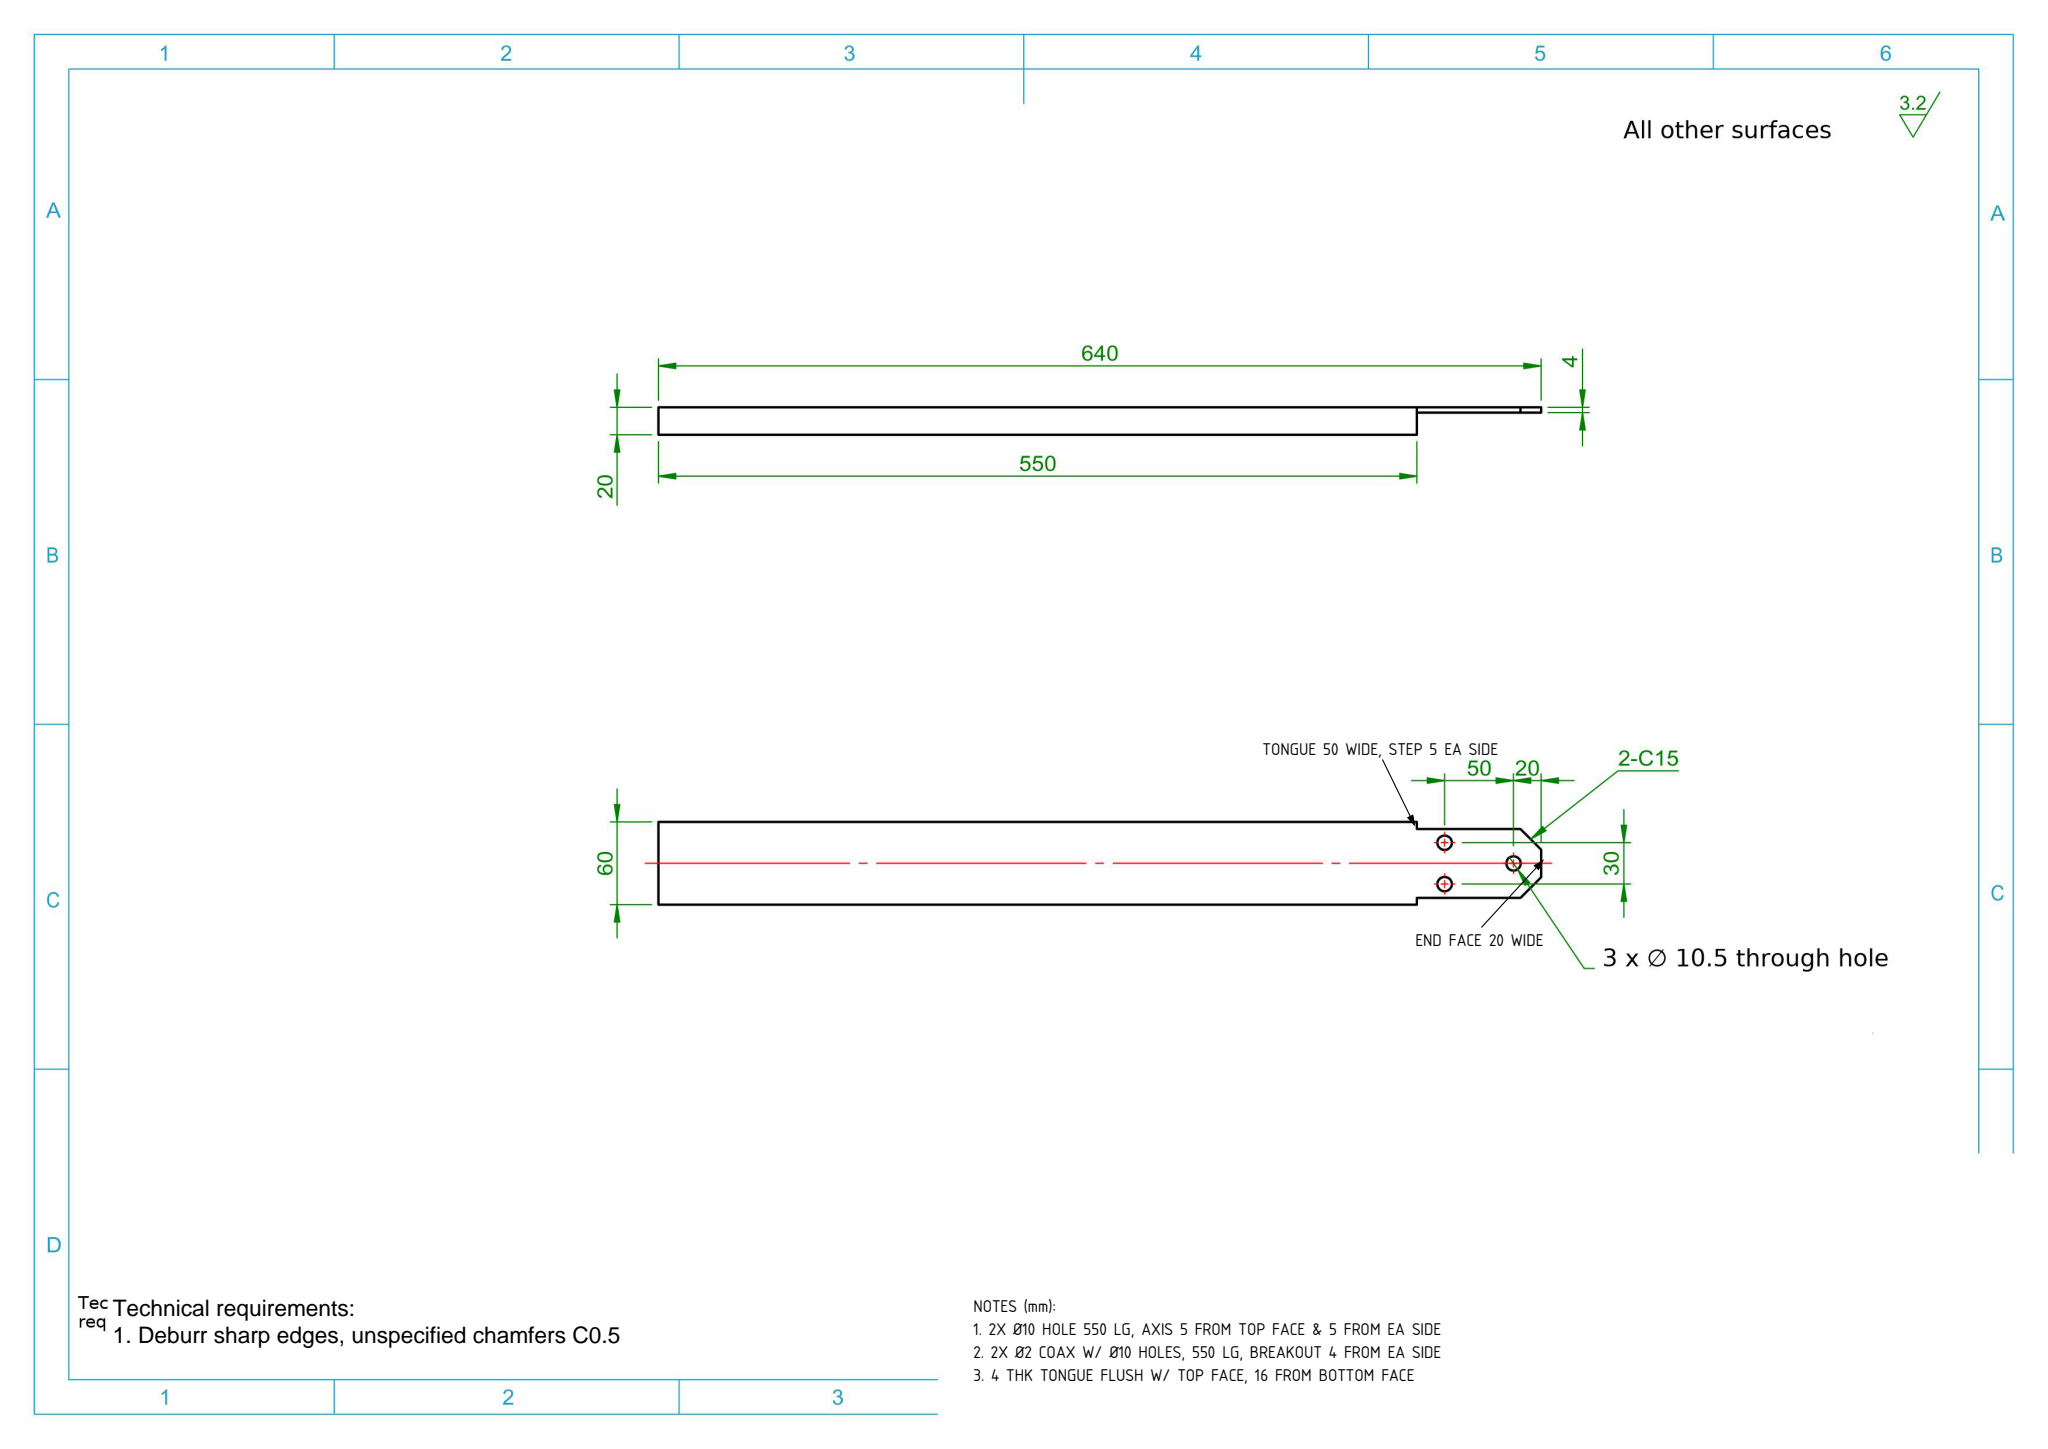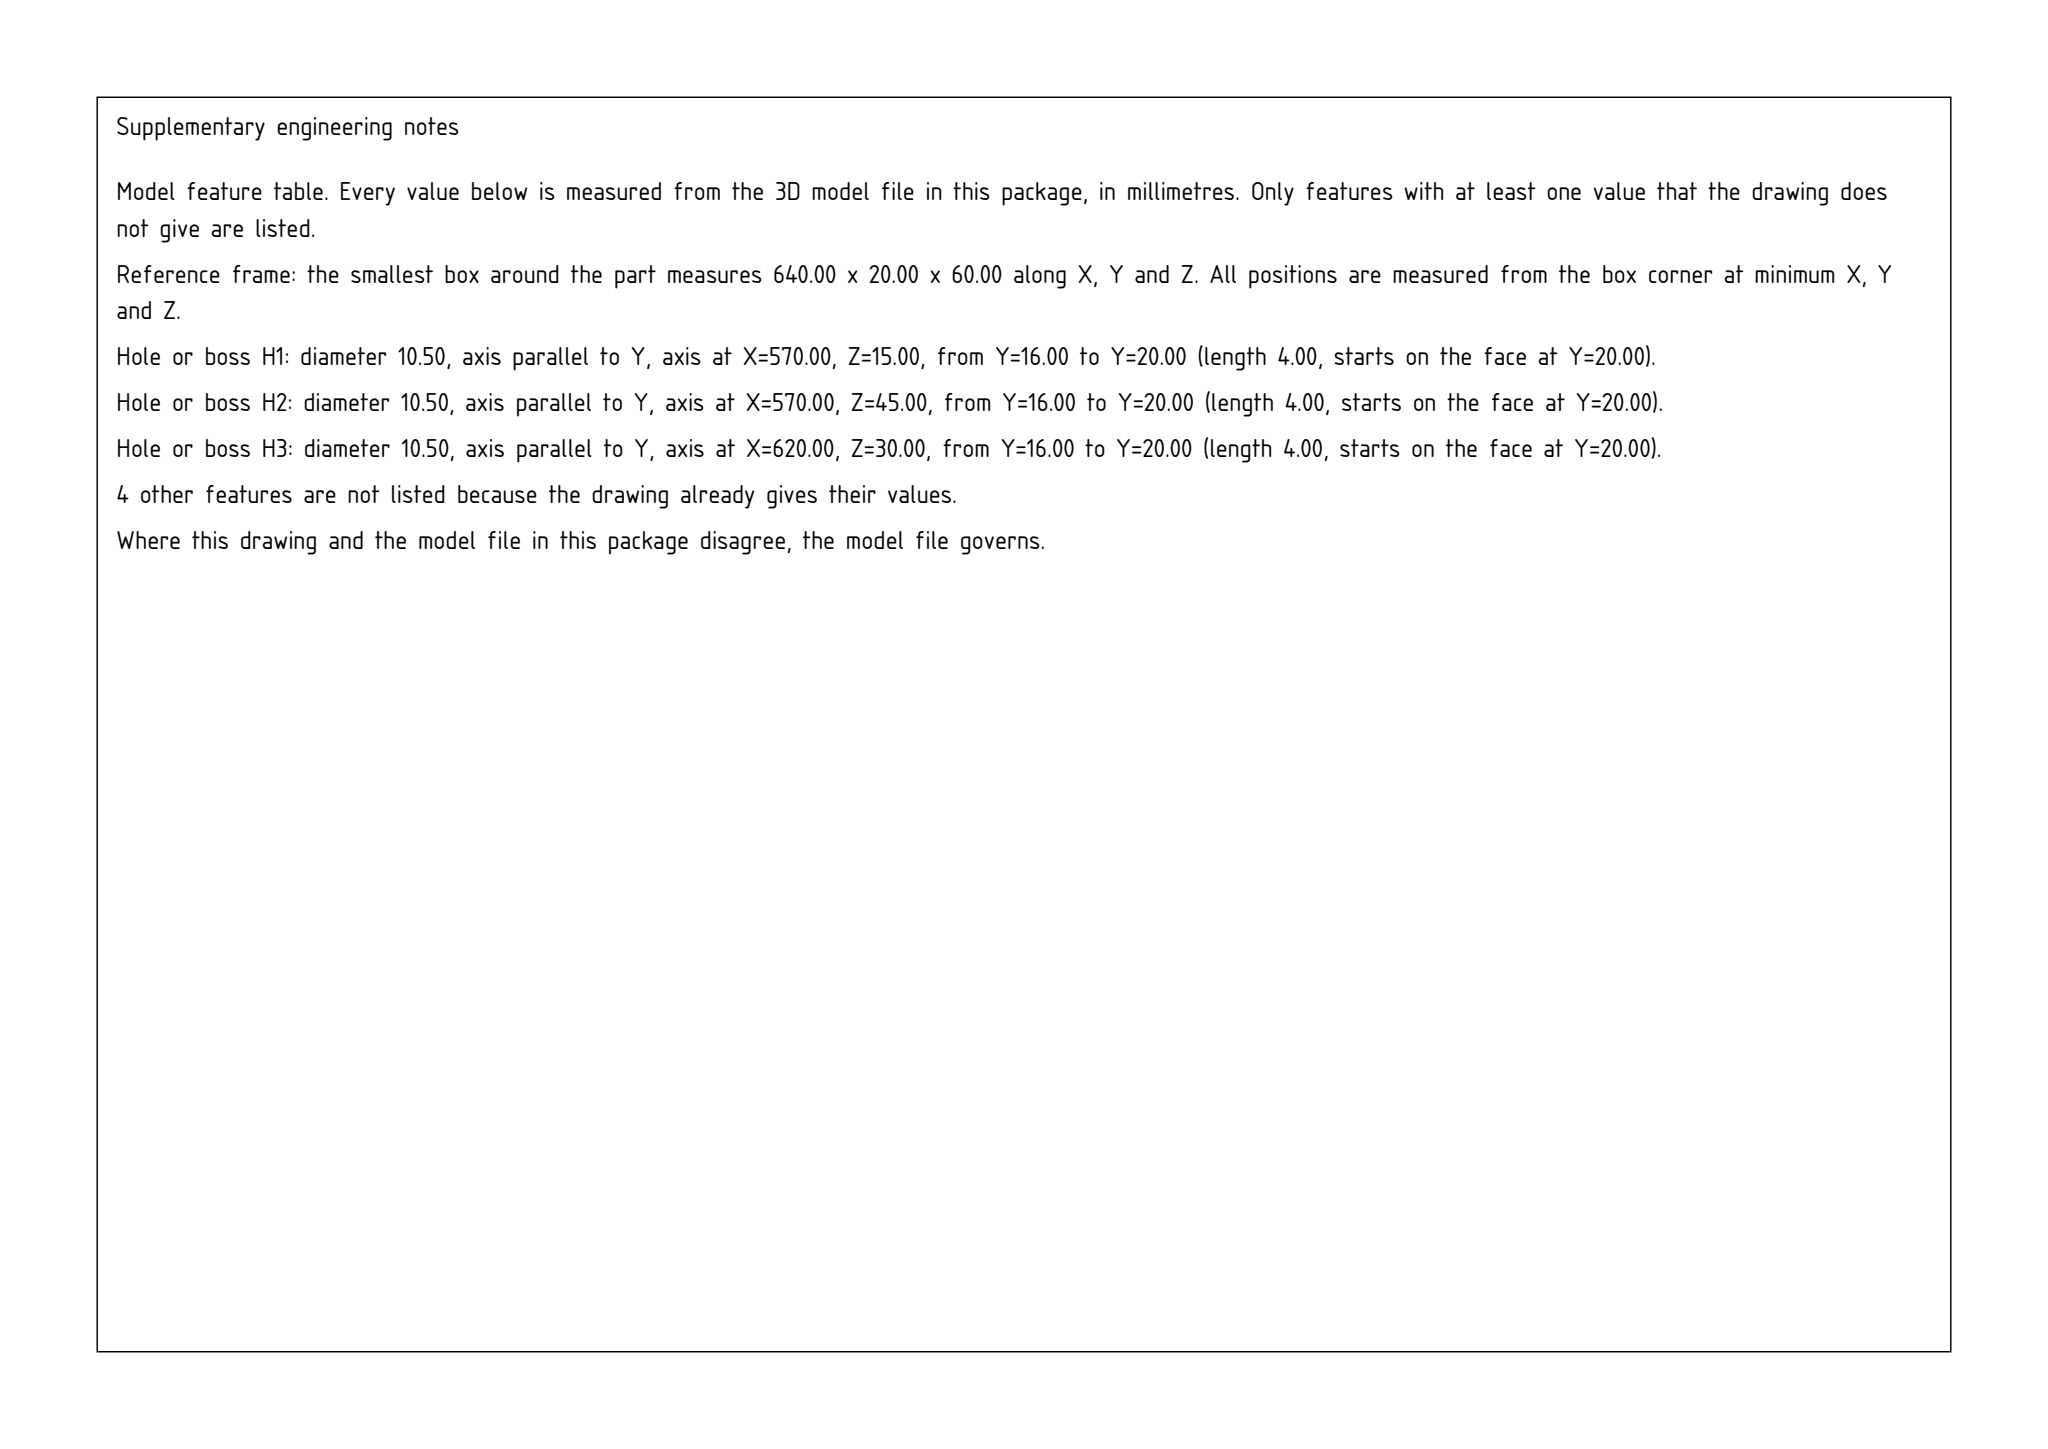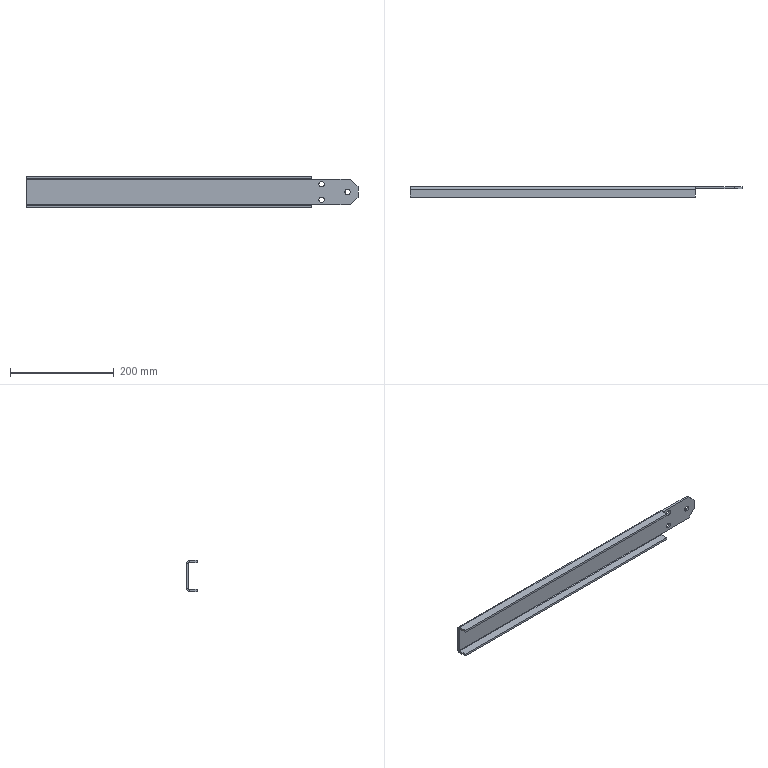Part | SolidWorks | mm | 1 solid | 32 faces | box 640 x 20 x 60 mm | volume 212795 mm3 | plane 22 | cylinder 10 | commonest cylinder face diameters 10.5 x6 10 x2 2 x2
Drawing notes:
TONGUE 50 WIDE (90 LG), STEP 5 DEEP EA SIDE, SYM ABT CL | from the solid: Tongue faces at z=5 and z=55 vs body z=0/60; step at x=550 to x=640
END FACE 20 WIDE AFTER 2-C15, SYM ABT CL | from the solid: 50 wide tongue less 2 x 15 chamfer = 20 at x=640 face
2X Ø10 HOLE 550 LG, AXIS 5 FROM TOP FACE & 5 FROM EA SIDE | from the solid: Ø10 cyl, axis x, y=15 (5 below top y=20), z=5 & z=55, length 550 from x=0
2X Ø2 COAX W/ Ø10 HOLES, 550 LG, BREAKOUT 4 FROM EA SIDE | from the solid: Ø2 cyl, axis x, y=15, z=5 & z=55, L=550; tangent planes z=4 and z=56
4 THK TONGUE FLUSH W/ TOP FACE, 16 FROM BOTTOM FACE | from the solid: y planes at 16 and 20; tongue y=16-20 within 20 thk
STEP:
#1=CARTESIAN_POINT('',(620.,16.,-35.25));
#2=VERTEX_POINT('',#1);
#3=CARTESIAN_POINT('',(620.,16.,-24.75));
#4=VERTEX_POINT('',#3);
#5=CARTESIAN_POINT('',(620.,16.,-30.));
#6=DIRECTION('',(-0.,1.,0.));
#7=DIRECTION('',(0.,0.,1.));
#8=AXIS2_PLACEMENT_3D('',#5,#6,#7);
#9=CIRCLE('',#8,5.25);
#10=EDGE_CURVE('',#2,#4,#9,.T.);
#11=ORIENTED_EDGE('',*,*,#10,.F.);
#12=CARTESIAN_POINT('',(620.,20.,-35.25));
#13=VERTEX_POINT('',#12);
#14=CARTESIAN_POINT('',(620.,20.,-35.25));
#15=DIRECTION('',(-0.,1.,0.));
#16=VECTOR('',#15,1000.);
#17=LINE('',#14,#16);
#18=EDGE_CURVE('',#2,#13,#17,.T.);
#19=ORIENTED_EDGE('',*,*,#18,.T.);
#20=CARTESIAN_POINT('',(620.,20.,-24.75));
#21=VERTEX_POINT('',#20);
#22=CARTESIAN_POINT('',(620.,20.,-30.));
#23=DIRECTION('',(-0.,1.,0.));
#24=DIRECTION('',(0.,0.,1.));
#25=AXIS2_PLACEMENT_3D('',#22,#23,#24);
#26=CIRCLE('',#25,5.25);
#27=EDGE_CURVE('',#13,#21,#26,.T.);
#28=ORIENTED_EDGE('',*,*,#27,.T.);
#29=CARTESIAN_POINT('',(620.,20.,-24.75));
#30=DIRECTION('',(-0.,1.,0.));
#31=VECTOR('',#30,1000.);
#32=LINE('',#29,#31);
#33=EDGE_CURVE('',#4,#21,#32,.T.);
#34=ORIENTED_EDGE('',*,*,#33,.F.);
#35=EDGE_LOOP('',(#11,#19,#28,#34));
#36=FACE_OUTER_BOUND('',#35,.T.);
#37=CARTESIAN_POINT('',(620.,20.,-30.));
#38=DIRECTION('',(-0.,1.,0.));
#39=DIRECTION('',(0.,0.,1.));
#40=AXIS2_PLACEMENT_3D('',#37,#38,#39);
#41=CYLINDRICAL_SURFACE('',#40,5.25);
#42=ADVANCED_FACE('',(#36),#41,.F.);
#43=CARTESIAN_POINT('',(570.,16.,-50.25));
#44=VERTEX_POINT('',#43);
#45=CARTESIAN_POINT('',(570.,16.,-39.75));
#46=VERTEX_POINT('',#45);
#47=CARTESIAN_POINT('',(570.,16.,-45.));
#48=DIRECTION('',(-0.,1.,0.));
#49=DIRECTION('',(0.,0.,1.));
#50=AXIS2_PLACEMENT_3D('',#47,#48,#49);
#51=CIRCLE('',#50,5.25);
#52=EDGE_CURVE('',#44,#46,#51,.T.);
#53=ORIENTED_EDGE('',*,*,#52,.F.);
#54=CARTESIAN_POINT('',(570.,20.,-50.25));
#55=VERTEX_POINT('',#54);
#56=CARTESIAN_POINT('',(570.,20.,-50.25));
#57=DIRECTION('',(-0.,1.,0.));
#58=VECTOR('',#57,1000.);
#59=LINE('',#56,#58);
#60=EDGE_CURVE('',#44,#55,#59,.T.);
#61=ORIENTED_EDGE('',*,*,#60,.T.);
#62=CARTESIAN_POINT('',(570.,20.,-39.75));
#63=VERTEX_POINT('',#62);
#64=CARTESIAN_POINT('',(570.,20.,-45.));
#65=DIRECTION('',(-0.,1.,0.));
#66=DIRECTION('',(0.,0.,1.));
#67=AXIS2_PLACEMENT_3D('',#64,#65,#66);
#68=CIRCLE('',#67,5.25);
#69=EDGE_CURVE('',#55,#63,#68,.T.);
#70=ORIENTED_EDGE('',*,*,#69,.T.);
#71=CARTESIAN_POINT('',(570.,20.,-39.75));
#72=DIRECTION('',(-0.,1.,0.));
#73=VECTOR('',#72,1000.);
#74=LINE('',#71,#73);
#75=EDGE_CURVE('',#46,#63,#74,.T.);
#76=ORIENTED_EDGE('',*,*,#75,.F.);
#77=EDGE_LOOP('',(#53,#61,#70,#76));
#78=FACE_OUTER_BOUND('',#77,.T.);
#79=CARTESIAN_POINT('',(570.,20.,-45.));
#80=DIRECTION('',(-0.,1.,0.));
#81=DIRECTION('',(0.,0.,1.));
#82=AXIS2_PLACEMENT_3D('',#79,#80,#81);
#83=CYLINDRICAL_SURFACE('',#82,5.25);
#84=ADVANCED_FACE('',(#78),#83,.F.);
#85=CARTESIAN_POINT('',(570.,16.,-20.25));
#86=VERTEX_POINT('',#85);
#87=CARTESIAN_POINT('',(570.,16.,-9.75));
#88=VERTEX_POINT('',#87);
#89=CARTESIAN_POINT('',(570.,16.,-15.));
#90=DIRECTION('',(-0.,1.,0.));
#91=DIRECTION('',(0.,0.,1.));
#92=AXIS2_PLACEMENT_3D('',#89,#90,#91);
#93=CIRCLE('',#92,5.25);
#94=EDGE_CURVE('',#86,#88,#93,.T.);
#95=ORIENTED_EDGE('',*,*,#94,.F.);
#96=CARTESIAN_POINT('',(570.,20.,-20.25));
#97=VERTEX_POINT('',#96);
#98=CARTESIAN_POINT('',(570.,20.,-20.25));
#99=DIRECTION('',(-0.,1.,0.));
#100=VECTOR('',#99,1000.);
#101=LINE('',#98,#100);
#102=EDGE_CURVE('',#86,#97,#101,.T.);
#103=ORIENTED_EDGE('',*,*,#102,.T.);
#104=CARTESIAN_POINT('',(570.,20.,-9.75));
#105=VERTEX_POINT('',#104);
#106=CARTESIAN_POINT('',(570.,20.,-15.));
#107=DIRECTION('',(-0.,1.,0.));
#108=DIRECTION('',(0.,0.,1.));
#109=AXIS2_PLACEMENT_3D('',#106,#107,#108);
#110=CIRCLE('',#109,5.25);
#111=EDGE_CURVE('',#97,#105,#110,.T.);
#112=ORIENTED_EDGE('',*,*,#111,.T.);
#113=CARTESIAN_POINT('',(570.,20.,-9.75));
#114=DIRECTION('',(-0.,1.,0.));
#115=VECTOR('',#114,1000.);
#116=LINE('',#113,#115);
#117=EDGE_CURVE('',#88,#105,#116,.T.);
#118=ORIENTED_EDGE('',*,*,#117,.F.);
#119=EDGE_LOOP('',(#95,#103,#112,#118));
#120=FACE_OUTER_BOUND('',#119,.T.);
#121=CARTESIAN_POINT('',(570.,20.,-15.));
#122=DIRECTION('',(-0.,1.,0.));
#123=DIRECTION('',(0.,0.,1.));
#124=AXIS2_PLACEMENT_3D('',#121,#122,#123);
#125=CYLINDRICAL_SURFACE('',#124,5.25);
#126=ADVANCED_FACE('',(#120),#125,.F.);
#127=CARTESIAN_POINT('',(550.,0.,-56.));
#128=VERTEX_POINT('',#127);
#129=CARTESIAN_POINT('',(550.,15.,-56.));
#130=VERTEX_POINT('',#129);
#131=CARTESIAN_POINT('',(550.,0.,-56.));
#132=DIRECTION('',(-0.,1.,0.));
#133=VECTOR('',#132,1000.);
#134=LINE('',#131,#133);
#135=EDGE_CURVE('',#128,#130,#134,.T.);
#136=ORIENTED_EDGE('',*,*,#135,.T.);
#137=CARTESIAN_POINT('',(0.,15.,-56.));
#138=VERTEX_POINT('',#137);
#139=CARTESIAN_POINT('',(640.,15.,-56.));
#140=DIRECTION('',(-1.,0.,0.));
#141=VECTOR('',#140,1000.);
#142=LINE('',#139,#141);
#143=EDGE_CURVE('',#130,#138,#142,.T.);
#144=ORIENTED_EDGE('',*,*,#143,.T.);
#145=CARTESIAN_POINT('',(0.,0.,-56.));
#146=VERTEX_POINT('',#145);
#147=CARTESIAN_POINT('',(0.,20.,-56.));
#148=DIRECTION('',(0.,-1.,-0.));
#149=VECTOR('',#148,1000.);
#150=LINE('',#147,#149);
#151=EDGE_CURVE('',#138,#146,#150,.T.);
#152=ORIENTED_EDGE('',*,*,#151,.T.);
#153=CARTESIAN_POINT('',(640.,0.,-56.));
#154=DIRECTION('',(-1.,0.,0.));
#155=VECTOR('',#154,1000.);
#156=LINE('',#153,#155);
#157=EDGE_CURVE('',#128,#146,#156,.T.);
#158=ORIENTED_EDGE('',*,*,#157,.F.);
#159=EDGE_LOOP('',(#136,#144,#152,#158));
#160=FACE_OUTER_BOUND('',#159,.T.);
#161=CARTESIAN_POINT('',(640.,20.,-56.));
#162=DIRECTION('',(-0.,-0.,-1.));
#163=DIRECTION('',(-1.,0.,0.));
#164=AXIS2_PLACEMENT_3D('',#161,#162,#163);
#165=PLANE('',#164);
#166=ADVANCED_FACE('',(#160),#165,.F.);
#167=CARTESIAN_POINT('',(550.,0.,-60.));
#168=VERTEX_POINT('',#167);
#169=CARTESIAN_POINT('',(0.,0.,-60.));
#170=VERTEX_POINT('',#169);
#171=CARTESIAN_POINT('',(640.,0.,-60.));
#172=DIRECTION('',(-1.,0.,0.));
#173=VECTOR('',#172,1000.);
#174=LINE('',#171,#173);
#175=EDGE_CURVE('',#168,#170,#174,.T.);
#176=ORIENTED_EDGE('',*,*,#175,.F.);
#177=CARTESIAN_POINT('',(550.,0.,-56.));
#178=DIRECTION('',(-0.,0.,1.));
#179=VECTOR('',#178,1000.);
#180=LINE('',#177,#179);
#181=EDGE_CURVE('',#168,#128,#180,.T.);
#182=ORIENTED_EDGE('',*,*,#181,.T.);
#183=ORIENTED_EDGE('',*,*,#157,.T.);
#184=CARTESIAN_POINT('',(0.,0.,-60.));
#185=DIRECTION('',(-0.,0.,1.));
#186=VECTOR('',#185,1000.);
#187=LINE('',#184,#186);
#188=EDGE_CURVE('',#170,#146,#187,.T.);
#189=ORIENTED_EDGE('',*,*,#188,.F.);
#190=EDGE_LOOP('',(#176,#182,#183,#189));
#191=FACE_OUTER_BOUND('',#190,.T.);
#192=CARTESIAN_POINT('',(640.,0.,-60.));
#193=DIRECTION('',(0.,-1.,0.));
#194=DIRECTION('',(0.,-0.,-1.));
#195=AXIS2_PLACEMENT_3D('',#192,#193,#194);
#196=PLANE('',#195);
#197=ADVANCED_FACE('',(#191),#196,.T.);
#198=CARTESIAN_POINT('',(550.,15.,-60.));
#199=VERTEX_POINT('',#198);
#200=CARTESIAN_POINT('',(0.,15.,-60.));
#201=VERTEX_POINT('',#200);
#202=CARTESIAN_POINT('',(640.,15.,-60.));
#203=DIRECTION('',(-1.,0.,0.));
#204=VECTOR('',#203,1000.);
#205=LINE('',#202,#204);
#206=EDGE_CURVE('',#199,#201,#205,.T.);
#207=ORIENTED_EDGE('',*,*,#206,.F.);
#208=CARTESIAN_POINT('',(550.,7.5,-60.));
#209=DIRECTION('',(-0.,1.,0.));
#210=VECTOR('',#209,1000.);
#211=LINE('',#208,#210);
#212=EDGE_CURVE('',#168,#199,#211,.T.);
#213=ORIENTED_EDGE('',*,*,#212,.F.);
#214=ORIENTED_EDGE('',*,*,#175,.T.);
#215=CARTESIAN_POINT('',(0.,20.,-60.));
#216=DIRECTION('',(0.,-1.,-0.));
#217=VECTOR('',#216,1000.);
#218=LINE('',#215,#217);
#219=EDGE_CURVE('',#201,#170,#218,.T.);
#220=ORIENTED_EDGE('',*,*,#219,.F.);
#221=EDGE_LOOP('',(#207,#213,#214,#220));
#222=FACE_OUTER_BOUND('',#221,.T.);
#223=CARTESIAN_POINT('',(640.,20.,-60.));
#224=DIRECTION('',(-0.,-0.,-1.));
#225=DIRECTION('',(-1.,0.,0.));
#226=AXIS2_PLACEMENT_3D('',#223,#224,#225);
#227=PLANE('',#226);
#228=ADVANCED_FACE('',(#222),#227,.T.);
#229=CARTESIAN_POINT('',(550.,20.,-55.));
#230=VERTEX_POINT('',#229);
#231=CARTESIAN_POINT('',(0.,20.,-55.));
#232=VERTEX_POINT('',#231);
#233=CARTESIAN_POINT('',(640.,20.,-55.));
#234=DIRECTION('',(-1.,0.,0.));
#235=VECTOR('',#234,1000.);
#236=LINE('',#233,#235);
#237=EDGE_CURVE('',#230,#232,#236,.T.);
#238=ORIENTED_EDGE('',*,*,#237,.F.);
#239=CARTESIAN_POINT('',(550.,15.,-55.));
#240=DIRECTION('',(-1.,0.,0.));
#241=DIRECTION('',(0.,0.,1.));
#242=AXIS2_PLACEMENT_3D('',#239,#240,#241);
#243=CIRCLE('',#242,5.);
#244=EDGE_CURVE('',#230,#199,#243,.T.);
#245=ORIENTED_EDGE('',*,*,#244,.T.);
#246=ORIENTED_EDGE('',*,*,#206,.T.);
#247=CARTESIAN_POINT('',(0.,15.,-55.));
#248=DIRECTION('',(-1.,0.,0.));
#249=DIRECTION('',(0.,0.,-1.));
#250=AXIS2_PLACEMENT_3D('',#247,#248,#249);
#251=CIRCLE('',#250,5.);
#252=EDGE_CURVE('',#232,#201,#251,.T.);
#253=ORIENTED_EDGE('',*,*,#252,.F.);
#254=EDGE_LOOP('',(#238,#245,#246,#253));
#255=FACE_OUTER_BOUND('',#254,.T.);
#256=CARTESIAN_POINT('',(640.,15.,-55.));
#257=DIRECTION('',(-1.,0.,0.));
#258=DIRECTION('',(0.,0.,1.));
#259=AXIS2_PLACEMENT_3D('',#256,#257,#258);
#260=CYLINDRICAL_SURFACE('',#259,5.);
#261=ADVANCED_FACE('',(#255),#260,.T.);
#262=CARTESIAN_POINT('',(550.,15.,-0.));
#263=VERTEX_POINT('',#262);
#264=CARTESIAN_POINT('',(0.,15.,0.));
#265=VERTEX_POINT('',#264);
#266=CARTESIAN_POINT('',(640.,15.,-0.));
#267=DIRECTION('',(-1.,0.,0.));
#268=VECTOR('',#267,1000.);
#269=LINE('',#266,#268);
#270=EDGE_CURVE('',#263,#265,#269,.T.);
#271=ORIENTED_EDGE('',*,*,#270,.F.);
#272=CARTESIAN_POINT('',(550.,20.,-5.));
#273=VERTEX_POINT('',#272);
#274=CARTESIAN_POINT('',(550.,15.,-5.));
#275=DIRECTION('',(-1.,0.,0.));
#276=DIRECTION('',(0.,0.,1.));
#277=AXIS2_PLACEMENT_3D('',#274,#275,#276);
#278=CIRCLE('',#277,5.);
#279=EDGE_CURVE('',#263,#273,#278,.T.);
#280=ORIENTED_EDGE('',*,*,#279,.T.);
#281=CARTESIAN_POINT('',(0.,20.,-5.));
#282=VERTEX_POINT('',#281);
#283=CARTESIAN_POINT('',(640.,20.,-5.));
#284=DIRECTION('',(-1.,0.,0.));
#285=VECTOR('',#284,1000.);
#286=LINE('',#283,#285);
#287=EDGE_CURVE('',#273,#282,#286,.T.);
#288=ORIENTED_EDGE('',*,*,#287,.T.);
#289=CARTESIAN_POINT('',(0.,15.,-5.));
#290=DIRECTION('',(-1.,0.,0.));
#291=DIRECTION('',(0.,0.,-1.));
#292=AXIS2_PLACEMENT_3D('',#289,#290,#291);
#293=CIRCLE('',#292,5.);
#294=EDGE_CURVE('',#265,#282,#293,.T.);
#295=ORIENTED_EDGE('',*,*,#294,.F.);
#296=EDGE_LOOP('',(#271,#280,#288,#295));
#297=FACE_OUTER_BOUND('',#296,.T.);
#298=CARTESIAN_POINT('',(640.,15.,-5.));
#299=DIRECTION('',(-1.,0.,0.));
#300=DIRECTION('',(0.,0.,1.));
#301=AXIS2_PLACEMENT_3D('',#298,#299,#300);
#302=CYLINDRICAL_SURFACE('',#301,5.);
#303=ADVANCED_FACE('',(#297),#302,.T.);
#304=CARTESIAN_POINT('',(550.,-0.,-0.));
#305=VERTEX_POINT('',#304);
#306=CARTESIAN_POINT('',(0.,0.,0.));
#307=VERTEX_POINT('',#306);
#308=CARTESIAN_POINT('',(640.,0.,-0.));
#309=DIRECTION('',(-1.,0.,0.));
#310=VECTOR('',#309,1000.);
#311=LINE('',#308,#310);
#312=EDGE_CURVE('',#305,#307,#311,.T.);
#313=ORIENTED_EDGE('',*,*,#312,.F.);
#314=CARTESIAN_POINT('',(550.,-0.,-0.));
#315=DIRECTION('',(-0.,1.,0.));
#316=VECTOR('',#315,1000.);
#317=LINE('',#314,#316);
#318=EDGE_CURVE('',#305,#263,#317,.T.);
#319=ORIENTED_EDGE('',*,*,#318,.T.);
#320=ORIENTED_EDGE('',*,*,#270,.T.);
#321=CARTESIAN_POINT('',(0.,0.,0.));
#322=DIRECTION('',(-0.,1.,0.));
#323=VECTOR('',#322,1000.);
#324=LINE('',#321,#323);
#325=EDGE_CURVE('',#307,#265,#324,.T.);
#326=ORIENTED_EDGE('',*,*,#325,.F.);
#327=EDGE_LOOP('',(#313,#319,#320,#326));
#328=FACE_OUTER_BOUND('',#327,.T.);
#329=CARTESIAN_POINT('',(640.,0.,-0.));
#330=DIRECTION('',(0.,0.,1.));
#331=DIRECTION('',(1.,-0.,-0.));
#332=AXIS2_PLACEMENT_3D('',#329,#330,#331);
#333=PLANE('',#332);
#334=ADVANCED_FACE('',(#328),#333,.T.);
#335=CARTESIAN_POINT('',(550.,0.,-4.));
#336=VERTEX_POINT('',#335);
#337=CARTESIAN_POINT('',(0.,0.,-4.));
#338=VERTEX_POINT('',#337);
#339=CARTESIAN_POINT('',(640.,0.,-4.));
#340=DIRECTION('',(-1.,0.,0.));
#341=VECTOR('',#340,1000.);
#342=LINE('',#339,#341);
#343=EDGE_CURVE('',#336,#338,#342,.T.);
#344=ORIENTED_EDGE('',*,*,#343,.F.);
#345=CARTESIAN_POINT('',(550.,-0.,-0.));
#346=DIRECTION('',(-0.,0.,1.));
#347=VECTOR('',#346,1000.);
#348=LINE('',#345,#347);
#349=EDGE_CURVE('',#336,#305,#348,.T.);
#350=ORIENTED_EDGE('',*,*,#349,.T.);
#351=ORIENTED_EDGE('',*,*,#312,.T.);
#352=CARTESIAN_POINT('',(0.,0.,-4.));
#353=DIRECTION('',(-0.,0.,1.));
#354=VECTOR('',#353,1000.);
#355=LINE('',#352,#354);
#356=EDGE_CURVE('',#338,#307,#355,.T.);
#357=ORIENTED_EDGE('',*,*,#356,.F.);
#358=EDGE_LOOP('',(#344,#350,#351,#357));
#359=FACE_OUTER_BOUND('',#358,.T.);
#360=CARTESIAN_POINT('',(640.,0.,-4.));
#361=DIRECTION('',(0.,-1.,0.));
#362=DIRECTION('',(0.,-0.,-1.));
#363=AXIS2_PLACEMENT_3D('',#360,#361,#362);
#364=PLANE('',#363);
#365=ADVANCED_FACE('',(#359),#364,.T.);
#366=CARTESIAN_POINT('',(550.,15.,-4.));
#367=VERTEX_POINT('',#366);
#368=CARTESIAN_POINT('',(550.,7.5,-4.));
#369=DIRECTION('',(-0.,1.,0.));
#370=VECTOR('',#369,1000.);
#371=LINE('',#368,#370);
#372=EDGE_CURVE('',#336,#367,#371,.T.);
#373=ORIENTED_EDGE('',*,*,#372,.F.);
#374=ORIENTED_EDGE('',*,*,#343,.T.);
#375=CARTESIAN_POINT('',(0.,15.,-4.));
#376=VERTEX_POINT('',#375);
#377=CARTESIAN_POINT('',(0.,0.,-4.));
#378=DIRECTION('',(-0.,1.,0.));
#379=VECTOR('',#378,1000.);
#380=LINE('',#377,#379);
#381=EDGE_CURVE('',#338,#376,#380,.T.);
#382=ORIENTED_EDGE('',*,*,#381,.T.);
#383=CARTESIAN_POINT('',(640.,15.,-4.));
#384=DIRECTION('',(-1.,0.,0.));
#385=VECTOR('',#384,1000.);
#386=LINE('',#383,#385);
#387=EDGE_CURVE('',#367,#376,#386,.T.);
#388=ORIENTED_EDGE('',*,*,#387,.F.);
#389=EDGE_LOOP('',(#373,#374,#382,#388));
#390=FACE_OUTER_BOUND('',#389,.T.);
#391=CARTESIAN_POINT('',(640.,0.,-4.));
#392=DIRECTION('',(0.,0.,1.));
#393=DIRECTION('',(1.,-0.,-0.));
#394=AXIS2_PLACEMENT_3D('',#391,#392,#393);
#395=PLANE('',#394);
#396=ADVANCED_FACE('',(#390),#395,.F.);
#397=CARTESIAN_POINT('',(550.,16.,-5.));
#398=VERTEX_POINT('',#397);
#399=CARTESIAN_POINT('',(550.,15.,-5.));
#400=DIRECTION('',(-1.,0.,0.));
#401=DIRECTION('',(0.,0.,-1.));
#402=AXIS2_PLACEMENT_3D('',#399,#400,#401);
#403=CIRCLE('',#402,1.);
#404=EDGE_CURVE('',#367,#398,#403,.T.);
#405=ORIENTED_EDGE('',*,*,#404,.F.);
#406=ORIENTED_EDGE('',*,*,#387,.T.);
#407=CARTESIAN_POINT('',(0.,16.,-5.));
#408=VERTEX_POINT('',#407);
#409=CARTESIAN_POINT('',(0.,15.,-5.));
#410=DIRECTION('',(-1.,0.,0.));
#411=DIRECTION('',(0.,0.,-1.));
#412=AXIS2_PLACEMENT_3D('',#409,#410,#411);
#413=CIRCLE('',#412,1.);
#414=EDGE_CURVE('',#376,#408,#413,.T.);
#415=ORIENTED_EDGE('',*,*,#414,.T.);
#416=CARTESIAN_POINT('',(640.,16.,-5.));
#417=DIRECTION('',(-1.,0.,0.));
#418=VECTOR('',#417,1000.);
#419=LINE('',#416,#418);
#420=EDGE_CURVE('',#398,#408,#419,.T.);
#421=ORIENTED_EDGE('',*,*,#420,.F.);
#422=EDGE_LOOP('',(#405,#406,#415,#421));
#423=FACE_OUTER_BOUND('',#422,.T.);
#424=CARTESIAN_POINT('',(640.,15.,-5.));
#425=DIRECTION('',(-1.,0.,0.));
#426=DIRECTION('',(0.,0.,1.));
#427=AXIS2_PLACEMENT_3D('',#424,#425,#426);
#428=CYLINDRICAL_SURFACE('',#427,1.);
#429=ADVANCED_FACE('',(#423),#428,.F.);
#430=CARTESIAN_POINT('',(550.,16.,-55.));
#431=VERTEX_POINT('',#430);
#432=CARTESIAN_POINT('',(550.,15.,-55.));
#433=DIRECTION('',(-1.,0.,0.));
#434=DIRECTION('',(0.,0.,1.));
#435=AXIS2_PLACEMENT_3D('',#432,#433,#434);
#436=CIRCLE('',#435,1.);
#437=EDGE_CURVE('',#431,#130,#436,.T.);
#438=ORIENTED_EDGE('',*,*,#437,.F.);
#439=CARTESIAN_POINT('',(0.,16.,-55.));
#440=VERTEX_POINT('',#439);
#441=CARTESIAN_POINT('',(640.,16.,-55.));
#442=DIRECTION('',(-1.,0.,0.));
#443=VECTOR('',#442,1000.);
#444=LINE('',#441,#443);
#445=EDGE_CURVE('',#431,#440,#444,.T.);
#446=ORIENTED_EDGE('',*,*,#445,.T.);
#447=CARTESIAN_POINT('',(0.,15.,-55.));
#448=DIRECTION('',(-1.,0.,0.));
#449=DIRECTION('',(0.,0.,-1.));
#450=AXIS2_PLACEMENT_3D('',#447,#448,#449);
#451=CIRCLE('',#450,1.);
#452=EDGE_CURVE('',#440,#138,#451,.T.);
#453=ORIENTED_EDGE('',*,*,#452,.T.);
#454=ORIENTED_EDGE('',*,*,#143,.F.);
#455=EDGE_LOOP('',(#438,#446,#453,#454));
#456=FACE_OUTER_BOUND('',#455,.T.);
#457=CARTESIAN_POINT('',(640.,15.,-55.));
#458=DIRECTION('',(-1.,0.,0.));
#459=DIRECTION('',(0.,0.,1.));
#460=AXIS2_PLACEMENT_3D('',#457,#458,#459);
#461=CYLINDRICAL_SURFACE('',#460,1.);
#462=ADVANCED_FACE('',(#456),#461,.F.);
#463=CARTESIAN_POINT('',(640.,20.,-20.));
#464=VERTEX_POINT('',#463);
#465=CARTESIAN_POINT('',(640.,20.,-40.));
#466=VERTEX_POINT('',#465);
#467=CARTESIAN_POINT('',(640.,20.,-0.));
#468=DIRECTION('',(0.,-0.,-1.));
#469=VECTOR('',#468,1000.);
#470=LINE('',#467,#469);
#471=EDGE_CURVE('',#464,#466,#470,.T.);
#472=ORIENTED_EDGE('',*,*,#471,.F.);
#473=CARTESIAN_POINT('',(640.,16.,-20.));
#474=VERTEX_POINT('',#473);
#475=CARTESIAN_POINT('',(640.,15.,-20.));
#476=DIRECTION('',(0.,-1.,-0.));
#477=VECTOR('',#476,1000.);
#478=LINE('',#475,#477);
#479=EDGE_CURVE('',#464,#474,#478,.T.);
#480=ORIENTED_EDGE('',*,*,#479,.T.);
#481=CARTESIAN_POINT('',(640.,16.,-40.));
#482=VERTEX_POINT('',#481);
#483=CARTESIAN_POINT('',(640.,16.,-0.));
#484=DIRECTION('',(0.,-0.,-1.));
#485=VECTOR('',#484,1000.);
#486=LINE('',#483,#485);
#487=EDGE_CURVE('',#474,#482,#486,.T.);
#488=ORIENTED_EDGE('',*,*,#487,.T.);
#489=CARTESIAN_POINT('',(640.,15.,-40.));
#490=DIRECTION('',(-0.,1.,0.));
#491=VECTOR('',#490,1000.);
#492=LINE('',#489,#491);
#493=EDGE_CURVE('',#482,#466,#492,.T.);
#494=ORIENTED_EDGE('',*,*,#493,.T.);
#495=EDGE_LOOP('',(#472,#480,#488,#494));
#496=FACE_OUTER_BOUND('',#495,.T.);
#497=CARTESIAN_POINT('',(640.,15.,-4.));
#498=DIRECTION('',(1.,-0.,0.));
#499=DIRECTION('',(0.,-0.,-1.));
#500=AXIS2_PLACEMENT_3D('',#497,#498,#499);
#501=PLANE('',#500);
#502=ADVANCED_FACE('',(#496),#501,.T.);
#503=CARTESIAN_POINT('',(0.,15.,0.));
#504=DIRECTION('',(0.,-0.,-1.));
#505=VECTOR('',#504,1000.);
#506=LINE('',#503,#505);
#507=EDGE_CURVE('',#265,#376,#506,.T.);
#508=ORIENTED_EDGE('',*,*,#507,.F.);
#509=ORIENTED_EDGE('',*,*,#294,.T.);
#510=CARTESIAN_POINT('',(0.,16.,-5.));
#511=DIRECTION('',(-0.,1.,0.));
#512=VECTOR('',#511,1000.);
#513=LINE('',#510,#512);
#514=EDGE_CURVE('',#408,#282,#513,.T.);
#515=ORIENTED_EDGE('',*,*,#514,.F.);
#516=ORIENTED_EDGE('',*,*,#414,.F.);
#517=EDGE_LOOP('',(#508,#509,#515,#516));
#518=FACE_OUTER_BOUND('',#517,.T.);
#519=CARTESIAN_POINT('',(0.,15.,0.));
#520=DIRECTION('',(-1.,0.,-0.));
#521=DIRECTION('',(-0.,0.,1.));
#522=AXIS2_PLACEMENT_3D('',#519,#520,#521);
#523=PLANE('',#522);
#524=ADVANCED_FACE('',(#518),#523,.T.);
#525=ORIENTED_EDGE('',*,*,#325,.T.);
#526=ORIENTED_EDGE('',*,*,#507,.T.);
#527=ORIENTED_EDGE('',*,*,#381,.F.);
#528=ORIENTED_EDGE('',*,*,#356,.T.);
#529=EDGE_LOOP('',(#525,#526,#527,#528));
#530=FACE_OUTER_BOUND('',#529,.T.);
#531=CARTESIAN_POINT('',(0.,16.,-5.));
#532=DIRECTION('',(-1.,0.,-0.));
#533=DIRECTION('',(-0.,0.,1.));
#534=AXIS2_PLACEMENT_3D('',#531,#532,#533);
#535=PLANE('',#534);
#536=ADVANCED_FACE('',(#530),#535,.T.);
#537=CARTESIAN_POINT('',(0.,20.,-55.));
#538=DIRECTION('',(0.,-1.,-0.));
#539=VECTOR('',#538,1000.);
#540=LINE('',#537,#539);
#541=EDGE_CURVE('',#232,#440,#540,.T.);
#542=ORIENTED_EDGE('',*,*,#541,.F.);
#543=ORIENTED_EDGE('',*,*,#252,.T.);
#544=CARTESIAN_POINT('',(0.,15.,-56.));
#545=DIRECTION('',(0.,-0.,-1.));
#546=VECTOR('',#545,1000.);
#547=LINE('',#544,#546);
#548=EDGE_CURVE('',#138,#201,#547,.T.);
#549=ORIENTED_EDGE('',*,*,#548,.F.);
#550=ORIENTED_EDGE('',*,*,#452,.F.);
#551=EDGE_LOOP('',(#542,#543,#549,#550));
#552=FACE_OUTER_BOUND('',#551,.T.);
#553=CARTESIAN_POINT('',(0.,20.,-55.));
#554=DIRECTION('',(-1.,0.,-0.));
#555=DIRECTION('',(-0.,0.,1.));
#556=AXIS2_PLACEMENT_3D('',#553,#554,#555);
#557=PLANE('',#556);
#558=ADVANCED_FACE('',(#552),#557,.T.);
#559=CARTESIAN_POINT('',(0.,20.,0.));
#560=DIRECTION('',(0.,-0.,-1.));
#561=VECTOR('',#560,1000.);
#562=LINE('',#559,#561);
#563=EDGE_CURVE('',#282,#232,#562,.T.);
#564=ORIENTED_EDGE('',*,*,#563,.T.);
#565=ORIENTED_EDGE('',*,*,#541,.T.);
#566=CARTESIAN_POINT('',(0.,16.,0.));
#567=DIRECTION('',(0.,-0.,-1.));
#568=VECTOR('',#567,1000.);
#569=LINE('',#566,#568);
#570=EDGE_CURVE('',#408,#440,#569,.T.);
#571=ORIENTED_EDGE('',*,*,#570,.F.);
#572=ORIENTED_EDGE('',*,*,#514,.T.);
#573=EDGE_LOOP('',(#564,#565,#571,#572));
#574=FACE_OUTER_BOUND('',#573,.T.);
#575=CARTESIAN_POINT('',(0.,15.,-56.));
#576=DIRECTION('',(-1.,0.,-0.));
#577=DIRECTION('',(-0.,0.,1.));
#578=AXIS2_PLACEMENT_3D('',#575,#576,#577);
#579=PLANE('',#578);
#580=ADVANCED_FACE('',(#574),#579,.T.);
#581=CARTESIAN_POINT('',(620.,20.,-30.));
#582=DIRECTION('',(-0.,1.,0.));
#583=DIRECTION('',(0.,0.,1.));
#584=AXIS2_PLACEMENT_3D('',#581,#582,#583);
#585=CIRCLE('',#584,5.25);
#586=EDGE_CURVE('',#21,#13,#585,.T.);
#587=ORIENTED_EDGE('',*,*,#586,.F.);
#588=ORIENTED_EDGE('',*,*,#27,.F.);
#589=EDGE_LOOP('',(#587,#588));
#590=FACE_BOUND('',#589,.T.);
#591=CARTESIAN_POINT('',(570.,20.,-45.));
#592=DIRECTION('',(-0.,1.,0.));
#593=DIRECTION('',(0.,0.,1.));
#594=AXIS2_PLACEMENT_3D('',#591,#592,#593);
#595=CIRCLE('',#594,5.25);
#596=EDGE_CURVE('',#63,#55,#595,.T.);
#597=ORIENTED_EDGE('',*,*,#596,.F.);
#598=ORIENTED_EDGE('',*,*,#69,.F.);
#599=EDGE_LOOP('',(#597,#598));
#600=FACE_BOUND('',#599,.T.);
#601=CARTESIAN_POINT('',(570.,20.,-15.));
#602=DIRECTION('',(-0.,1.,0.));
#603=DIRECTION('',(0.,0.,1.));
#604=AXIS2_PLACEMENT_3D('',#601,#602,#603);
#605=CIRCLE('',#604,5.25);
#606=EDGE_CURVE('',#105,#97,#605,.T.);
#607=ORIENTED_EDGE('',*,*,#606,.F.);
#608=ORIENTED_EDGE('',*,*,#111,.F.);
#609=EDGE_LOOP('',(#607,#608));
#610=FACE_BOUND('',#609,.T.);
#611=CARTESIAN_POINT('',(625.,20.,-5.));
#612=VERTEX_POINT('',#611);
#613=CARTESIAN_POINT('',(640.,20.,-5.));
#614=DIRECTION('',(-1.,0.,0.));
#615=VECTOR('',#614,1000.);
#616=LINE('',#613,#615);
#617=EDGE_CURVE('',#612,#273,#616,.T.);
#618=ORIENTED_EDGE('',*,*,#617,.F.);
#619=CARTESIAN_POINT('',(630.,20.,-10.));
#620=DIRECTION('',(0.7071,-0.,-0.7071));
#621=VECTOR('',#620,1000.);
#622=LINE('',#619,#621);
#623=EDGE_CURVE('',#612,#464,#622,.T.);
#624=ORIENTED_EDGE('',*,*,#623,.T.);
#625=ORIENTED_EDGE('',*,*,#471,.T.);
#626=CARTESIAN_POINT('',(625.,20.,-55.));
#627=VERTEX_POINT('',#626);
#628=CARTESIAN_POINT('',(660.,20.,-20.));
#629=DIRECTION('',(-0.7071,0.,-0.7071));
#630=VECTOR('',#629,1000.);
#631=LINE('',#628,#630);
#632=EDGE_CURVE('',#466,#627,#631,.T.);
#633=ORIENTED_EDGE('',*,*,#632,.T.);
#634=CARTESIAN_POINT('',(640.,20.,-55.));
#635=DIRECTION('',(-1.,0.,0.));
#636=VECTOR('',#635,1000.);
#637=LINE('',#634,#636);
#638=EDGE_CURVE('',#627,#230,#637,.T.);
#639=ORIENTED_EDGE('',*,*,#638,.T.);
#640=ORIENTED_EDGE('',*,*,#237,.T.);
#641=ORIENTED_EDGE('',*,*,#563,.F.);
#642=ORIENTED_EDGE('',*,*,#287,.F.);
#643=EDGE_LOOP('',(#618,#624,#625,#633,#639,#640,#641,#642));
#644=FACE_OUTER_BOUND('',#643,.T.);
#645=CARTESIAN_POINT('',(640.,20.,-0.));
#646=DIRECTION('',(-0.,1.,-0.));
#647=DIRECTION('',(-0.,0.,1.));
#648=AXIS2_PLACEMENT_3D('',#645,#646,#647);
#649=PLANE('',#648);
#650=ADVANCED_FACE('',(#590,#600,#610,#644),#649,.T.);
#651=CARTESIAN_POINT('',(620.,16.,-30.));
#652=DIRECTION('',(-0.,1.,0.));
#653=DIRECTION('',(0.,0.,1.));
#654=AXIS2_PLACEMENT_3D('',#651,#652,#653);
#655=CIRCLE('',#654,5.25);
#656=EDGE_CURVE('',#4,#2,#655,.T.);
#657=ORIENTED_EDGE('',*,*,#656,.T.);
#658=ORIENTED_EDGE('',*,*,#10,.T.);
#659=EDGE_LOOP('',(#657,#658));
#660=FACE_BOUND('',#659,.T.);
#661=CARTESIAN_POINT('',(570.,16.,-45.));
#662=DIRECTION('',(-0.,1.,0.));
#663=DIRECTION('',(0.,0.,1.));
#664=AXIS2_PLACEMENT_3D('',#661,#662,#663);
#665=CIRCLE('',#664,5.25);
#666=EDGE_CURVE('',#46,#44,#665,.T.);
#667=ORIENTED_EDGE('',*,*,#666,.T.);
#668=ORIENTED_EDGE('',*,*,#52,.T.);
#669=EDGE_LOOP('',(#667,#668));
#670=FACE_BOUND('',#669,.T.);
#671=CARTESIAN_POINT('',(570.,16.,-15.));
#672=DIRECTION('',(-0.,1.,0.));
#673=DIRECTION('',(0.,0.,1.));
#674=AXIS2_PLACEMENT_3D('',#671,#672,#673);
#675=CIRCLE('',#674,5.25);
#676=EDGE_CURVE('',#88,#86,#675,.T.);
#677=ORIENTED_EDGE('',*,*,#676,.T.);
#678=ORIENTED_EDGE('',*,*,#94,.T.);
#679=EDGE_LOOP('',(#677,#678));
#680=FACE_BOUND('',#679,.T.);
#681=ORIENTED_EDGE('',*,*,#487,.F.);
#682=CARTESIAN_POINT('',(625.,16.,-5.));
#683=VERTEX_POINT('',#682);
#684=CARTESIAN_POINT('',(640.,16.,-20.));
#685=DIRECTION('',(-0.7071,0.,0.7071));
#686=VECTOR('',#685,1000.);
#687=LINE('',#684,#686);
#688=EDGE_CURVE('',#474,#683,#687,.T.);
#689=ORIENTED_EDGE('',*,*,#688,.T.);
#690=CARTESIAN_POINT('',(640.,16.,-5.));
#691=DIRECTION('',(-1.,0.,0.));
#692=VECTOR('',#691,1000.);
#693=LINE('',#690,#692);
#694=EDGE_CURVE('',#683,#398,#693,.T.);
#695=ORIENTED_EDGE('',*,*,#694,.T.);
#696=ORIENTED_EDGE('',*,*,#420,.T.);
#697=ORIENTED_EDGE('',*,*,#570,.T.);
#698=ORIENTED_EDGE('',*,*,#445,.F.);
#699=CARTESIAN_POINT('',(625.,16.,-55.));
#700=VERTEX_POINT('',#699);
#701=CARTESIAN_POINT('',(640.,16.,-55.));
#702=DIRECTION('',(-1.,0.,0.));
#703=VECTOR('',#702,1000.);
#704=LINE('',#701,#703);
#705=EDGE_CURVE('',#700,#431,#704,.T.);
#706=ORIENTED_EDGE('',*,*,#705,.F.);
#707=CARTESIAN_POINT('',(640.,16.,-40.));
#708=DIRECTION('',(0.7071,-0.,0.7071));
#709=VECTOR('',#708,1000.);
#710=LINE('',#707,#709);
#711=EDGE_CURVE('',#700,#482,#710,.T.);
#712=ORIENTED_EDGE('',*,*,#711,.T.);
#713=EDGE_LOOP('',(#681,#689,#695,#696,#697,#698,#706,#712));
#714=FACE_OUTER_BOUND('',#713,.T.);
#715=CARTESIAN_POINT('',(640.,16.,-0.));
#716=DIRECTION('',(-0.,1.,-0.));
#717=DIRECTION('',(-0.,0.,1.));
#718=AXIS2_PLACEMENT_3D('',#715,#716,#717);
#719=PLANE('',#718);
#720=ADVANCED_FACE('',(#660,#670,#680,#714),#719,.F.);
#721=ORIENTED_EDGE('',*,*,#151,.F.);
#722=ORIENTED_EDGE('',*,*,#548,.T.);
#723=ORIENTED_EDGE('',*,*,#219,.T.);
#724=ORIENTED_EDGE('',*,*,#188,.T.);
#725=EDGE_LOOP('',(#721,#722,#723,#724));
#726=FACE_OUTER_BOUND('',#725,.T.);
#727=CARTESIAN_POINT('',(0.,15.,-55.));
#728=DIRECTION('',(1.,-0.,0.));
#729=DIRECTION('',(0.,-0.,-1.));
#730=AXIS2_PLACEMENT_3D('',#727,#728,#729);
#731=PLANE('',#730);
#732=ADVANCED_FACE('',(#726),#731,.F.);
#733=CARTESIAN_POINT('',(550.,16.,-55.));
#734=DIRECTION('',(-0.,1.,0.));
#735=VECTOR('',#734,1000.);
#736=LINE('',#733,#735);
#737=EDGE_CURVE('',#431,#230,#736,.T.);
#738=ORIENTED_EDGE('',*,*,#737,.F.);
#739=ORIENTED_EDGE('',*,*,#437,.T.);
#740=CARTESIAN_POINT('',(550.,15.,-60.));
#741=DIRECTION('',(-0.,0.,1.));
#742=VECTOR('',#741,1000.);
#743=LINE('',#740,#742);
#744=EDGE_CURVE('',#199,#130,#743,.T.);
#745=ORIENTED_EDGE('',*,*,#744,.F.);
#746=ORIENTED_EDGE('',*,*,#244,.F.);
#747=EDGE_LOOP('',(#738,#739,#745,#746));
#748=FACE_OUTER_BOUND('',#747,.T.);
#749=CARTESIAN_POINT('',(550.,15.,-55.));
#750=DIRECTION('',(1.,-0.,0.));
#751=DIRECTION('',(0.,-0.,-1.));
#752=AXIS2_PLACEMENT_3D('',#749,#750,#751);
#753=PLANE('',#752);
#754=ADVANCED_FACE('',(#748),#753,.T.);
#755=ORIENTED_EDGE('',*,*,#638,.F.);
#756=CARTESIAN_POINT('',(625.,16.,-55.));
#757=DIRECTION('',(0.,-1.,-0.));
#758=VECTOR('',#757,1000.);
#759=LINE('',#756,#758);
#760=EDGE_CURVE('',#627,#700,#759,.T.);
#761=ORIENTED_EDGE('',*,*,#760,.T.);
#762=ORIENTED_EDGE('',*,*,#705,.T.);
#763=ORIENTED_EDGE('',*,*,#737,.T.);
#764=EDGE_LOOP('',(#755,#761,#762,#763));
#765=FACE_OUTER_BOUND('',#764,.T.);
#766=CARTESIAN_POINT('',(595.,16.,-55.));
#767=DIRECTION('',(-0.,-0.,-1.));
#768=DIRECTION('',(-1.,0.,0.));
#769=AXIS2_PLACEMENT_3D('',#766,#767,#768);
#770=PLANE('',#769);
#771=ADVANCED_FACE('',(#765),#770,.T.);
#772=ORIENTED_EDGE('',*,*,#212,.T.);
#773=ORIENTED_EDGE('',*,*,#744,.T.);
#774=ORIENTED_EDGE('',*,*,#135,.F.);
#775=ORIENTED_EDGE('',*,*,#181,.F.);
#776=EDGE_LOOP('',(#772,#773,#774,#775));
#777=FACE_OUTER_BOUND('',#776,.T.);
#778=CARTESIAN_POINT('',(550.,0.,-56.));
#779=DIRECTION('',(-1.,-0.,0.));
#780=DIRECTION('',(-0.,1.,0.));
#781=AXIS2_PLACEMENT_3D('',#778,#779,#780);
#782=PLANE('',#781);
#783=ADVANCED_FACE('',(#777),#782,.F.);
#784=CARTESIAN_POINT('',(550.,15.,-0.));
#785=DIRECTION('',(0.,-0.,-1.));
#786=VECTOR('',#785,1000.);
#787=LINE('',#784,#786);
#788=EDGE_CURVE('',#263,#367,#787,.T.);
#789=ORIENTED_EDGE('',*,*,#788,.T.);
#790=ORIENTED_EDGE('',*,*,#404,.T.);
#791=CARTESIAN_POINT('',(550.,16.,-5.));
#792=DIRECTION('',(-0.,1.,0.));
#793=VECTOR('',#792,1000.);
#794=LINE('',#791,#793);
#795=EDGE_CURVE('',#398,#273,#794,.T.);
#796=ORIENTED_EDGE('',*,*,#795,.T.);
#797=ORIENTED_EDGE('',*,*,#279,.F.);
#798=EDGE_LOOP('',(#789,#790,#796,#797));
#799=FACE_OUTER_BOUND('',#798,.T.);
#800=CARTESIAN_POINT('',(550.,15.,-5.));
#801=DIRECTION('',(1.,-0.,0.));
#802=DIRECTION('',(0.,-0.,-1.));
#803=AXIS2_PLACEMENT_3D('',#800,#801,#802);
#804=PLANE('',#803);
#805=ADVANCED_FACE('',(#799),#804,.T.);
#806=ORIENTED_EDGE('',*,*,#694,.F.);
#807=CARTESIAN_POINT('',(625.,16.,-5.));
#808=DIRECTION('',(-0.,1.,0.));
#809=VECTOR('',#808,1000.);
#810=LINE('',#807,#809);
#811=EDGE_CURVE('',#683,#612,#810,.T.);
#812=ORIENTED_EDGE('',*,*,#811,.T.);
#813=ORIENTED_EDGE('',*,*,#617,.T.);
#814=ORIENTED_EDGE('',*,*,#795,.F.);
#815=EDGE_LOOP('',(#806,#812,#813,#814));
#816=FACE_OUTER_BOUND('',#815,.T.);
#817=CARTESIAN_POINT('',(595.,16.,-5.));
#818=DIRECTION('',(-0.,-0.,-1.));
#819=DIRECTION('',(-1.,0.,0.));
#820=AXIS2_PLACEMENT_3D('',#817,#818,#819);
#821=PLANE('',#820);
#822=ADVANCED_FACE('',(#816),#821,.F.);
#823=ORIENTED_EDGE('',*,*,#349,.F.);
#824=ORIENTED_EDGE('',*,*,#372,.T.);
#825=ORIENTED_EDGE('',*,*,#788,.F.);
#826=ORIENTED_EDGE('',*,*,#318,.F.);
#827=EDGE_LOOP('',(#823,#824,#825,#826));
#828=FACE_OUTER_BOUND('',#827,.T.);
#829=CARTESIAN_POINT('',(550.,-0.,-0.));
#830=DIRECTION('',(-1.,-0.,0.));
#831=DIRECTION('',(-0.,1.,0.));
#832=AXIS2_PLACEMENT_3D('',#829,#830,#831);
#833=PLANE('',#832);
#834=ADVANCED_FACE('',(#828),#833,.F.);
#835=ORIENTED_EDGE('',*,*,#623,.F.);
#836=ORIENTED_EDGE('',*,*,#811,.F.);
#837=ORIENTED_EDGE('',*,*,#688,.F.);
#838=ORIENTED_EDGE('',*,*,#479,.F.);
#839=EDGE_LOOP('',(#835,#836,#837,#838));
#840=FACE_OUTER_BOUND('',#839,.T.);
#841=CARTESIAN_POINT('',(640.,15.,-20.));
#842=DIRECTION('',(0.7071,0.,0.7071));
#843=DIRECTION('',(-0.,1.,0.));
#844=AXIS2_PLACEMENT_3D('',#841,#842,#843);
#845=PLANE('',#844);
#846=ADVANCED_FACE('',(#840),#845,.T.);
#847=ORIENTED_EDGE('',*,*,#711,.F.);
#848=ORIENTED_EDGE('',*,*,#760,.F.);
#849=ORIENTED_EDGE('',*,*,#632,.F.);
#850=ORIENTED_EDGE('',*,*,#493,.F.);
#851=EDGE_LOOP('',(#847,#848,#849,#850));
#852=FACE_OUTER_BOUND('',#851,.T.);
#853=CARTESIAN_POINT('',(640.,15.,-40.));
#854=DIRECTION('',(-0.7071,-0.,0.7071));
#855=DIRECTION('',(-0.,1.,0.));
#856=AXIS2_PLACEMENT_3D('',#853,#854,#855);
#857=PLANE('',#856);
#858=ADVANCED_FACE('',(#852),#857,.F.);
#859=ORIENTED_EDGE('',*,*,#102,.F.);
#860=ORIENTED_EDGE('',*,*,#676,.F.);
#861=ORIENTED_EDGE('',*,*,#117,.T.);
#862=ORIENTED_EDGE('',*,*,#606,.T.);
#863=EDGE_LOOP('',(#859,#860,#861,#862));
#864=FACE_OUTER_BOUND('',#863,.T.);
#865=CARTESIAN_POINT('',(570.,20.,-15.));
#866=DIRECTION('',(-0.,1.,0.));
#867=DIRECTION('',(0.,0.,1.));
#868=AXIS2_PLACEMENT_3D('',#865,#866,#867);
#869=CYLINDRICAL_SURFACE('',#868,5.25);
#870=ADVANCED_FACE('',(#864),#869,.F.);
#871=ORIENTED_EDGE('',*,*,#60,.F.);
#872=ORIENTED_EDGE('',*,*,#666,.F.);
#873=ORIENTED_EDGE('',*,*,#75,.T.);
#874=ORIENTED_EDGE('',*,*,#596,.T.);
#875=EDGE_LOOP('',(#871,#872,#873,#874));
#876=FACE_OUTER_BOUND('',#875,.T.);
#877=CARTESIAN_POINT('',(570.,20.,-45.));
#878=DIRECTION('',(-0.,1.,0.));
#879=DIRECTION('',(0.,0.,1.));
#880=AXIS2_PLACEMENT_3D('',#877,#878,#879);
#881=CYLINDRICAL_SURFACE('',#880,5.25);
#882=ADVANCED_FACE('',(#876),#881,.F.);
#883=ORIENTED_EDGE('',*,*,#18,.F.);
#884=ORIENTED_EDGE('',*,*,#656,.F.);
#885=ORIENTED_EDGE('',*,*,#33,.T.);
#886=ORIENTED_EDGE('',*,*,#586,.T.);
#887=EDGE_LOOP('',(#883,#884,#885,#886));
#888=FACE_OUTER_BOUND('',#887,.T.);
#889=CARTESIAN_POINT('',(620.,20.,-30.));
#890=DIRECTION('',(-0.,1.,0.));
#891=DIRECTION('',(0.,0.,1.));
#892=AXIS2_PLACEMENT_3D('',#889,#890,#891);
#893=CYLINDRICAL_SURFACE('',#892,5.25);
#894=ADVANCED_FACE('',(#888),#893,.F.);
#895=CLOSED_SHELL('',(#42,#84,#126,#166,#197,#228,#261,#303,#334,#365,#396,#429,#462,#502,#524,#536,#558,#580,#650,#720,#732,#754,#771,#783,#805,#822,#834,#846,#858,#870,#882,#894));
#896=MANIFOLD_SOLID_BREP('',#895);
#897=CARTESIAN_POINT('',(0.,0.,0.));
#898=DIRECTION('',(0.,0.,1.));
#899=DIRECTION('',(1.,0.,0.));
#900=AXIS2_PLACEMENT_3D('',#897,#898,#899);
#901=(LENGTH_UNIT()NAMED_UNIT(*)SI_UNIT(.MILLI.,.METRE.));
#902=UNCERTAINTY_MEASURE_WITH_UNIT(LENGTH_MEASURE(0.00001),#901,'','');
#903=(NAMED_UNIT(*)PLANE_ANGLE_UNIT()SI_UNIT($,.RADIAN.));
#904=(NAMED_UNIT(*)SI_UNIT($,.STERADIAN.)SOLID_ANGLE_UNIT());
#905=(GEOMETRIC_REPRESENTATION_CONTEXT(3)GLOBAL_UNCERTAINTY_ASSIGNED_CONTEXT((#902))GLOBAL_UNIT_ASSIGNED_CONTEXT((#901,#903,#904))REPRESENTATION_CONTEXT('',''));
#906=ADVANCED_BREP_SHAPE_REPRESENTATION('',(#896,#900),#905);